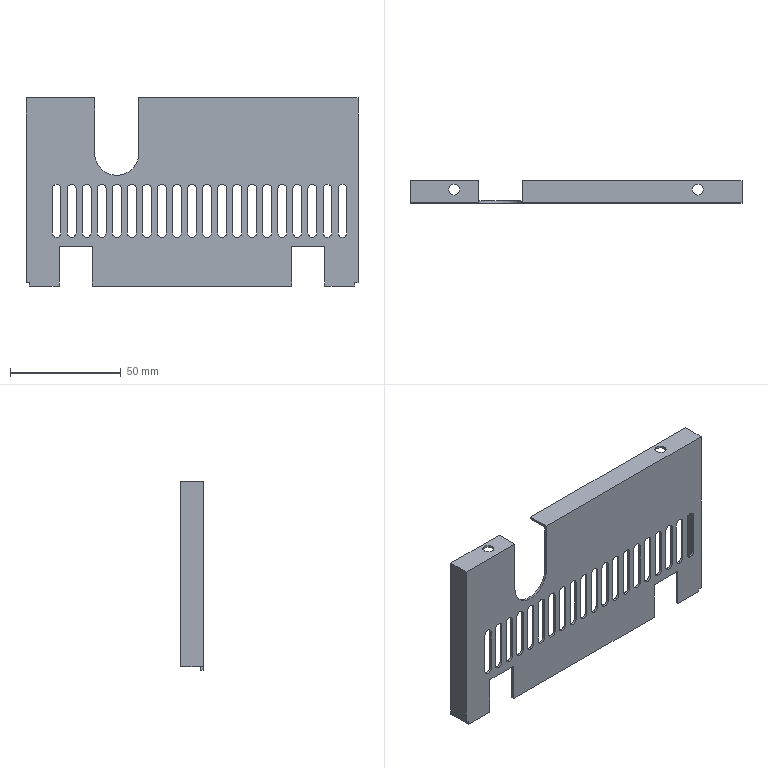Component | NX | REAR_PANEL | 1 solid | 110 faces | volume 12313 mm3 | plane 67 | cylinder 43 | commonest cylinder face diameters 4 x40 5 x2 20 x1